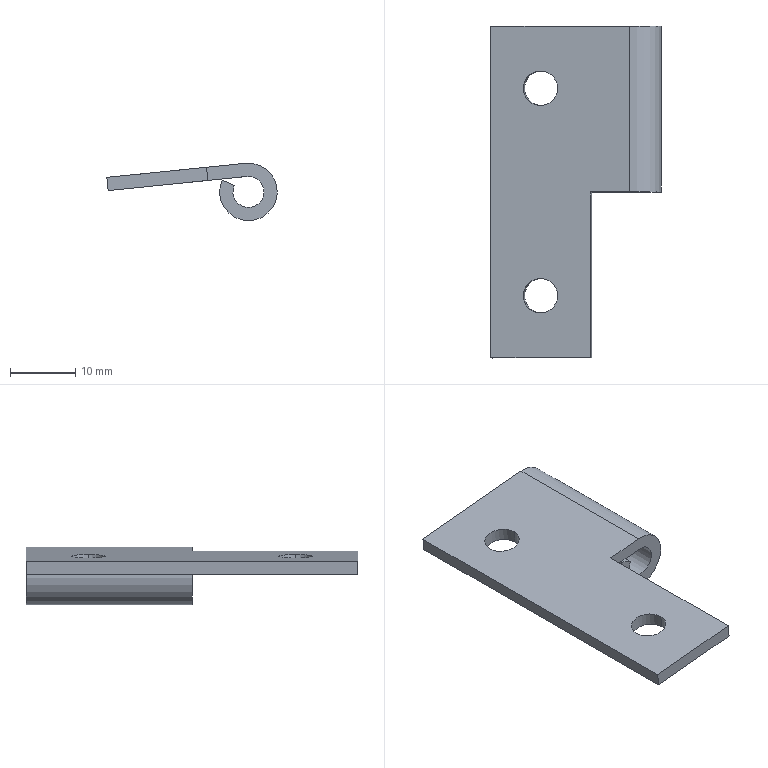Component | SolidWorks | Imported3-1 | 1 solid | 15 faces | box 26.08 x 50.8 x 8.81 mm | volume 2720 mm3 | plane 9 | cylinder 6 | commonest cylinder face diameters 5.283 x4 8.814 x1 4.75 x1
STEP:
#1=COLOUR_RGB('',0.7922,0.8196,0.9333);
#2=FILL_AREA_STYLE_COLOUR('',#1);
#3=FILL_AREA_STYLE('',(#2));
#4=SURFACE_STYLE_FILL_AREA(#3);
#5=SURFACE_SIDE_STYLE('',(#4));
#6=SURFACE_STYLE_USAGE(.BOTH.,#5);
#7=PRESENTATION_STYLE_ASSIGNMENT((#6));
#8=CARTESIAN_POINT('',(-8.855,6.998,9.99));
#9=VERTEX_POINT('',#8);
#10=CARTESIAN_POINT('',(-8.648,6.998,10.011));
#11=VERTEX_POINT('',#10);
#12=CARTESIAN_POINT('',(-8.751,6.998,10.001));
#13=DIRECTION('',(0.1012,0.,-0.9949));
#14=DIRECTION('',(-0.9949,0.,-0.1012));
#15=AXIS2_PLACEMENT_3D('',#12,#13,#14);
#16=CIRCLE('',#15,0.104);
#17=EDGE_CURVE('',#9,#11,#16,.T.);
#18=ORIENTED_EDGE('',*,*,#17,.F.);
#19=CARTESIAN_POINT('',(-8.847,6.998,9.91));
#20=VERTEX_POINT('',#19);
#21=CARTESIAN_POINT('',(-8.855,6.998,9.99));
#22=DIRECTION('',(0.1012,0.,-0.9949));
#23=VECTOR('',#22,39.37);
#24=LINE('',#21,#23);
#25=EDGE_CURVE('',#9,#20,#24,.T.);
#26=ORIENTED_EDGE('',*,*,#25,.T.);
#27=CARTESIAN_POINT('',(-8.64,6.998,9.931));
#28=VERTEX_POINT('',#27);
#29=CARTESIAN_POINT('',(-8.743,6.998,9.921));
#30=DIRECTION('',(0.1012,0.,-0.9949));
#31=DIRECTION('',(-0.9949,0.,-0.1012));
#32=AXIS2_PLACEMENT_3D('',#29,#30,#31);
#33=CIRCLE('',#32,0.104);
#34=EDGE_CURVE('',#20,#28,#33,.T.);
#35=ORIENTED_EDGE('',*,*,#34,.T.);
#36=CARTESIAN_POINT('',(-8.648,6.998,10.011));
#37=DIRECTION('',(0.1012,0.,-0.9949));
#38=VECTOR('',#37,39.37);
#39=LINE('',#36,#38);
#40=EDGE_CURVE('',#11,#28,#39,.T.);
#41=ORIENTED_EDGE('',*,*,#40,.F.);
#42=EDGE_LOOP('',(#18,#26,#35,#41));
#43=FACE_OUTER_BOUND('',#42,.T.);
#44=CARTESIAN_POINT('',(-8.751,6.998,10.001));
#45=DIRECTION('',(0.1012,0.,-0.9949));
#46=DIRECTION('',(0.9949,0.,0.1012));
#47=AXIS2_PLACEMENT_3D('',#44,#45,#46);
#48=CYLINDRICAL_SURFACE('',#47,0.104);
#49=ADVANCED_FACE('',(#43),#48,.F.);
#50=CARTESIAN_POINT('',(-8.855,5.748,9.99));
#51=VERTEX_POINT('',#50);
#52=CARTESIAN_POINT('',(-8.648,5.748,10.011));
#53=VERTEX_POINT('',#52);
#54=CARTESIAN_POINT('',(-8.751,5.748,10.001));
#55=DIRECTION('',(0.1012,0.,-0.9949));
#56=DIRECTION('',(0.9949,0.,0.1012));
#57=AXIS2_PLACEMENT_3D('',#54,#55,#56);
#58=CIRCLE('',#57,0.104);
#59=EDGE_CURVE('',#51,#53,#58,.T.);
#60=ORIENTED_EDGE('',*,*,#59,.F.);
#61=CARTESIAN_POINT('',(-8.847,5.748,9.91));
#62=VERTEX_POINT('',#61);
#63=CARTESIAN_POINT('',(-8.855,5.748,9.99));
#64=DIRECTION('',(0.1012,0.,-0.9949));
#65=VECTOR('',#64,39.37);
#66=LINE('',#63,#65);
#67=EDGE_CURVE('',#51,#62,#66,.T.);
#68=ORIENTED_EDGE('',*,*,#67,.T.);
#69=CARTESIAN_POINT('',(-8.64,5.748,9.931));
#70=VERTEX_POINT('',#69);
#71=CARTESIAN_POINT('',(-8.743,5.748,9.921));
#72=DIRECTION('',(0.1012,0.,-0.9949));
#73=DIRECTION('',(0.9949,0.,0.1012));
#74=AXIS2_PLACEMENT_3D('',#71,#72,#73);
#75=CIRCLE('',#74,0.104);
#76=EDGE_CURVE('',#62,#70,#75,.T.);
#77=ORIENTED_EDGE('',*,*,#76,.T.);
#78=CARTESIAN_POINT('',(-8.648,5.748,10.011));
#79=DIRECTION('',(0.1012,0.,-0.9949));
#80=VECTOR('',#79,39.37);
#81=LINE('',#78,#80);
#82=EDGE_CURVE('',#53,#70,#81,.T.);
#83=ORIENTED_EDGE('',*,*,#82,.F.);
#84=EDGE_LOOP('',(#60,#68,#77,#83));
#85=FACE_OUTER_BOUND('',#84,.T.);
#86=CARTESIAN_POINT('',(-8.751,5.748,10.001));
#87=DIRECTION('',(0.1012,0.,-0.9949));
#88=DIRECTION('',(0.9949,0.,0.1012));
#89=AXIS2_PLACEMENT_3D('',#86,#87,#88);
#90=CYLINDRICAL_SURFACE('',#89,0.104);
#91=ADVANCED_FACE('',(#85),#90,.F.);
#92=CARTESIAN_POINT('',(-9.05,5.373,9.97));
#93=VERTEX_POINT('',#92);
#94=CARTESIAN_POINT('',(-9.05,7.373,9.97));
#95=VERTEX_POINT('',#94);
#96=CARTESIAN_POINT('',(-9.05,5.373,9.97));
#97=DIRECTION('',(-0.,1.,0.));
#98=VECTOR('',#97,39.37);
#99=LINE('',#96,#98);
#100=EDGE_CURVE('',#93,#95,#99,.T.);
#101=ORIENTED_EDGE('',*,*,#100,.T.);
#102=CARTESIAN_POINT('',(-9.042,7.373,9.891));
#103=VERTEX_POINT('',#102);
#104=CARTESIAN_POINT('',(-9.042,7.373,9.891));
#105=DIRECTION('',(-0.1012,-0.,0.9949));
#106=VECTOR('',#105,39.37);
#107=LINE('',#104,#106);
#108=EDGE_CURVE('',#103,#95,#107,.T.);
#109=ORIENTED_EDGE('',*,*,#108,.F.);
#110=CARTESIAN_POINT('',(-9.042,5.373,9.891));
#111=VERTEX_POINT('',#110);
#112=CARTESIAN_POINT('',(-9.042,5.373,9.891));
#113=DIRECTION('',(-0.,1.,0.));
#114=VECTOR('',#113,39.37);
#115=LINE('',#112,#114);
#116=EDGE_CURVE('',#111,#103,#115,.T.);
#117=ORIENTED_EDGE('',*,*,#116,.F.);
#118=CARTESIAN_POINT('',(-9.042,5.373,9.891));
#119=DIRECTION('',(-0.1012,-0.,0.9949));
#120=VECTOR('',#119,39.37);
#121=LINE('',#118,#120);
#122=EDGE_CURVE('',#111,#93,#121,.T.);
#123=ORIENTED_EDGE('',*,*,#122,.T.);
#124=EDGE_LOOP('',(#101,#109,#117,#123));
#125=FACE_OUTER_BOUND('',#124,.T.);
#126=CARTESIAN_POINT('',(-9.042,5.373,9.891));
#127=DIRECTION('',(0.9949,0.,0.1012));
#128=DIRECTION('',(-0.1012,-0.,0.9949));
#129=AXIS2_PLACEMENT_3D('',#126,#127,#128);
#130=PLANE('',#129);
#131=ADVANCED_FACE('',(#125),#130,.F.);
#132=CARTESIAN_POINT('',(-8.214,7.373,10.055));
#133=VERTEX_POINT('',#132);
#134=CARTESIAN_POINT('',(-9.05,7.373,9.97));
#135=DIRECTION('',(0.9949,0.,0.1012));
#136=VECTOR('',#135,39.37);
#137=LINE('',#134,#136);
#138=EDGE_CURVE('',#95,#133,#137,.T.);
#139=ORIENTED_EDGE('',*,*,#138,.T.);
#140=CARTESIAN_POINT('',(-8.206,7.373,9.976));
#141=VERTEX_POINT('',#140);
#142=CARTESIAN_POINT('',(-8.206,7.373,9.976));
#143=DIRECTION('',(-0.1012,-0.,0.9949));
#144=VECTOR('',#143,39.37);
#145=LINE('',#142,#144);
#146=EDGE_CURVE('',#141,#133,#145,.T.);
#147=ORIENTED_EDGE('',*,*,#146,.F.);
#148=CARTESIAN_POINT('',(-9.042,7.373,9.891));
#149=DIRECTION('',(0.9949,0.,0.1012));
#150=VECTOR('',#149,39.37);
#151=LINE('',#148,#150);
#152=EDGE_CURVE('',#103,#141,#151,.T.);
#153=ORIENTED_EDGE('',*,*,#152,.F.);
#154=ORIENTED_EDGE('',*,*,#108,.T.);
#155=EDGE_LOOP('',(#139,#147,#153,#154));
#156=FACE_OUTER_BOUND('',#155,.T.);
#157=CARTESIAN_POINT('',(-9.042,7.373,9.891));
#158=DIRECTION('',(0.,-1.,-0.));
#159=DIRECTION('',(0.1012,0.,-0.9949));
#160=AXIS2_PLACEMENT_3D('',#157,#158,#159);
#161=PLANE('',#160);
#162=ADVANCED_FACE('',(#156),#161,.F.);
#163=CARTESIAN_POINT('',(-8.441,5.373,9.952));
#164=VERTEX_POINT('',#163);
#165=CARTESIAN_POINT('',(-9.042,5.373,9.891));
#166=DIRECTION('',(-0.9949,-0.,-0.1012));
#167=VECTOR('',#166,39.37);
#168=LINE('',#165,#167);
#169=EDGE_CURVE('',#164,#111,#168,.T.);
#170=ORIENTED_EDGE('',*,*,#169,.F.);
#171=CARTESIAN_POINT('',(-8.449,5.373,10.031));
#172=VERTEX_POINT('',#171);
#173=CARTESIAN_POINT('',(-8.414,5.373,9.686));
#174=DIRECTION('',(-0.1012,-0.,0.9949));
#175=VECTOR('',#174,39.37);
#176=LINE('',#173,#175);
#177=EDGE_CURVE('',#164,#172,#176,.T.);
#178=ORIENTED_EDGE('',*,*,#177,.T.);
#179=CARTESIAN_POINT('',(-9.05,5.373,9.97));
#180=DIRECTION('',(-0.9949,-0.,-0.1012));
#181=VECTOR('',#180,39.37);
#182=LINE('',#179,#181);
#183=EDGE_CURVE('',#172,#93,#182,.T.);
#184=ORIENTED_EDGE('',*,*,#183,.T.);
#185=ORIENTED_EDGE('',*,*,#122,.F.);
#186=EDGE_LOOP('',(#170,#178,#184,#185));
#187=FACE_OUTER_BOUND('',#186,.T.);
#188=CARTESIAN_POINT('',(-9.042,5.373,9.891));
#189=DIRECTION('',(-0.,1.,0.));
#190=DIRECTION('',(-0.1012,-0.,0.9949));
#191=AXIS2_PLACEMENT_3D('',#188,#189,#190);
#192=PLANE('',#191);
#193=ADVANCED_FACE('',(#187),#192,.F.);
#194=CARTESIAN_POINT('',(-8.743,6.998,9.921));
#195=DIRECTION('',(0.1012,0.,-0.9949));
#196=DIRECTION('',(-0.9949,0.,-0.1012));
#197=AXIS2_PLACEMENT_3D('',#194,#195,#196);
#198=CIRCLE('',#197,0.104);
#199=EDGE_CURVE('',#28,#20,#198,.T.);
#200=ORIENTED_EDGE('',*,*,#199,.F.);
#201=ORIENTED_EDGE('',*,*,#34,.F.);
#202=EDGE_LOOP('',(#200,#201));
#203=FACE_BOUND('',#202,.T.);
#204=CARTESIAN_POINT('',(-8.743,5.748,9.921));
#205=DIRECTION('',(0.1012,0.,-0.9949));
#206=DIRECTION('',(0.9949,0.,0.1012));
#207=AXIS2_PLACEMENT_3D('',#204,#205,#206);
#208=CIRCLE('',#207,0.104);
#209=EDGE_CURVE('',#70,#62,#208,.T.);
#210=ORIENTED_EDGE('',*,*,#209,.F.);
#211=ORIENTED_EDGE('',*,*,#76,.F.);
#212=EDGE_LOOP('',(#210,#211));
#213=FACE_BOUND('',#212,.T.);
#214=CARTESIAN_POINT('',(-8.441,6.373,9.952));
#215=VERTEX_POINT('',#214);
#216=CARTESIAN_POINT('',(-8.441,7.373,9.952));
#217=DIRECTION('',(-0.,1.,0.));
#218=VECTOR('',#217,39.37);
#219=LINE('',#216,#218);
#220=EDGE_CURVE('',#164,#215,#219,.T.);
#221=ORIENTED_EDGE('',*,*,#220,.F.);
#222=ORIENTED_EDGE('',*,*,#169,.T.);
#223=ORIENTED_EDGE('',*,*,#116,.T.);
#224=ORIENTED_EDGE('',*,*,#152,.T.);
#225=CARTESIAN_POINT('',(-8.206,6.373,9.976));
#226=VERTEX_POINT('',#225);
#227=CARTESIAN_POINT('',(-8.206,5.373,9.976));
#228=DIRECTION('',(0.,-1.,-0.));
#229=VECTOR('',#228,39.37);
#230=LINE('',#227,#229);
#231=EDGE_CURVE('',#141,#226,#230,.T.);
#232=ORIENTED_EDGE('',*,*,#231,.T.);
#233=CARTESIAN_POINT('',(-9.042,6.373,9.891));
#234=DIRECTION('',(0.9949,0.,0.1012));
#235=VECTOR('',#234,39.37);
#236=LINE('',#233,#235);
#237=EDGE_CURVE('',#215,#226,#236,.T.);
#238=ORIENTED_EDGE('',*,*,#237,.F.);
#239=EDGE_LOOP('',(#221,#222,#223,#224,#232,#238));
#240=FACE_OUTER_BOUND('',#239,.T.);
#241=CARTESIAN_POINT('',(-9.042,7.373,9.891));
#242=DIRECTION('',(0.1012,0.,-0.9949));
#243=DIRECTION('',(0.9949,0.,0.1012));
#244=AXIS2_PLACEMENT_3D('',#241,#242,#243);
#245=PLANE('',#244);
#246=ADVANCED_FACE('',(#203,#213,#240),#245,.T.);
#247=CARTESIAN_POINT('',(-8.751,6.998,10.001));
#248=DIRECTION('',(0.1012,0.,-0.9949));
#249=DIRECTION('',(-0.9949,0.,-0.1012));
#250=AXIS2_PLACEMENT_3D('',#247,#248,#249);
#251=CIRCLE('',#250,0.104);
#252=EDGE_CURVE('',#11,#9,#251,.T.);
#253=ORIENTED_EDGE('',*,*,#252,.T.);
#254=ORIENTED_EDGE('',*,*,#17,.T.);
#255=EDGE_LOOP('',(#253,#254));
#256=FACE_BOUND('',#255,.T.);
#257=CARTESIAN_POINT('',(-8.751,5.748,10.001));
#258=DIRECTION('',(0.1012,0.,-0.9949));
#259=DIRECTION('',(0.9949,0.,0.1012));
#260=AXIS2_PLACEMENT_3D('',#257,#258,#259);
#261=CIRCLE('',#260,0.104);
#262=EDGE_CURVE('',#53,#51,#261,.T.);
#263=ORIENTED_EDGE('',*,*,#262,.T.);
#264=ORIENTED_EDGE('',*,*,#59,.T.);
#265=EDGE_LOOP('',(#263,#264));
#266=FACE_BOUND('',#265,.T.);
#267=ORIENTED_EDGE('',*,*,#183,.F.);
#268=CARTESIAN_POINT('',(-8.449,6.373,10.031));
#269=VERTEX_POINT('',#268);
#270=CARTESIAN_POINT('',(-8.449,5.373,10.031));
#271=DIRECTION('',(0.,-1.,-0.));
#272=VECTOR('',#271,39.37);
#273=LINE('',#270,#272);
#274=EDGE_CURVE('',#269,#172,#273,.T.);
#275=ORIENTED_EDGE('',*,*,#274,.F.);
#276=CARTESIAN_POINT('',(-8.214,6.373,10.055));
#277=VERTEX_POINT('',#276);
#278=CARTESIAN_POINT('',(-8.041,6.373,10.073));
#279=DIRECTION('',(-0.9949,-0.,-0.1012));
#280=VECTOR('',#279,39.37);
#281=LINE('',#278,#280);
#282=EDGE_CURVE('',#277,#269,#281,.T.);
#283=ORIENTED_EDGE('',*,*,#282,.F.);
#284=CARTESIAN_POINT('',(-8.214,5.373,10.055));
#285=DIRECTION('',(0.,-1.,-0.));
#286=VECTOR('',#285,39.37);
#287=LINE('',#284,#286);
#288=EDGE_CURVE('',#133,#277,#287,.T.);
#289=ORIENTED_EDGE('',*,*,#288,.F.);
#290=ORIENTED_EDGE('',*,*,#138,.F.);
#291=ORIENTED_EDGE('',*,*,#100,.F.);
#292=EDGE_LOOP('',(#267,#275,#283,#289,#290,#291));
#293=FACE_OUTER_BOUND('',#292,.T.);
#294=CARTESIAN_POINT('',(-9.05,7.373,9.97));
#295=DIRECTION('',(0.1012,0.,-0.9949));
#296=DIRECTION('',(0.9949,0.,0.1012));
#297=AXIS2_PLACEMENT_3D('',#294,#295,#296);
#298=PLANE('',#297);
#299=ADVANCED_FACE('',(#256,#266,#293),#298,.F.);
#300=CARTESIAN_POINT('',(-8.282,6.373,9.921));
#301=VERTEX_POINT('',#300);
#302=CARTESIAN_POINT('',(-8.355,6.373,9.954));
#303=VERTEX_POINT('',#302);
#304=CARTESIAN_POINT('',(-8.282,6.373,9.921));
#305=DIRECTION('',(-0.9122,-0.,0.4098));
#306=VECTOR('',#305,39.37);
#307=LINE('',#304,#306);
#308=EDGE_CURVE('',#301,#303,#307,.T.);
#309=ORIENTED_EDGE('',*,*,#308,.F.);
#310=CARTESIAN_POINT('',(-8.282,7.373,9.921));
#311=VERTEX_POINT('',#310);
#312=CARTESIAN_POINT('',(-8.282,5.373,9.921));
#313=DIRECTION('',(0.,-1.,-0.));
#314=VECTOR('',#313,39.37);
#315=LINE('',#312,#314);
#316=EDGE_CURVE('',#311,#301,#315,.T.);
#317=ORIENTED_EDGE('',*,*,#316,.F.);
#318=CARTESIAN_POINT('',(-8.355,7.373,9.954));
#319=VERTEX_POINT('',#318);
#320=CARTESIAN_POINT('',(-8.282,7.373,9.921));
#321=DIRECTION('',(-0.9122,-0.,0.4098));
#322=VECTOR('',#321,39.37);
#323=LINE('',#320,#322);
#324=EDGE_CURVE('',#311,#319,#323,.T.);
#325=ORIENTED_EDGE('',*,*,#324,.T.);
#326=CARTESIAN_POINT('',(-8.355,5.373,9.954));
#327=DIRECTION('',(0.,-1.,-0.));
#328=VECTOR('',#327,39.37);
#329=LINE('',#326,#328);
#330=EDGE_CURVE('',#319,#303,#329,.T.);
#331=ORIENTED_EDGE('',*,*,#330,.T.);
#332=EDGE_LOOP('',(#309,#317,#325,#331));
#333=FACE_OUTER_BOUND('',#332,.T.);
#334=CARTESIAN_POINT('',(-8.282,6.373,9.921));
#335=DIRECTION('',(-0.4098,0.,-0.9122));
#336=DIRECTION('',(0.,-1.,-0.));
#337=AXIS2_PLACEMENT_3D('',#334,#335,#336);
#338=PLANE('',#337);
#339=ADVANCED_FACE('',(#333),#338,.F.);
#340=ORIENTED_EDGE('',*,*,#324,.F.);
#341=CARTESIAN_POINT('',(-8.196,7.373,9.883));
#342=DIRECTION('',(-0.,1.,0.));
#343=DIRECTION('',(0.1012,0.,-0.9949));
#344=AXIS2_PLACEMENT_3D('',#341,#342,#343);
#345=CIRCLE('',#344,0.0935);
#346=EDGE_CURVE('',#141,#311,#345,.T.);
#347=ORIENTED_EDGE('',*,*,#346,.F.);
#348=ORIENTED_EDGE('',*,*,#146,.T.);
#349=CARTESIAN_POINT('',(-8.196,7.373,9.883));
#350=DIRECTION('',(-0.,1.,0.));
#351=DIRECTION('',(0.1012,0.,-0.9949));
#352=AXIS2_PLACEMENT_3D('',#349,#350,#351);
#353=CIRCLE('',#352,0.1735);
#354=EDGE_CURVE('',#133,#319,#353,.T.);
#355=ORIENTED_EDGE('',*,*,#354,.T.);
#356=EDGE_LOOP('',(#340,#347,#348,#355));
#357=FACE_OUTER_BOUND('',#356,.T.);
#358=CARTESIAN_POINT('',(-8.196,7.373,9.883));
#359=DIRECTION('',(-0.,1.,0.));
#360=DIRECTION('',(-0.1012,-0.,0.9949));
#361=AXIS2_PLACEMENT_3D('',#358,#359,#360);
#362=PLANE('',#361);
#363=ADVANCED_FACE('',(#357),#362,.T.);
#364=CARTESIAN_POINT('',(-8.196,6.373,9.883));
#365=DIRECTION('',(0.,-1.,-0.));
#366=DIRECTION('',(0.9949,0.,0.1012));
#367=AXIS2_PLACEMENT_3D('',#364,#365,#366);
#368=CIRCLE('',#367,0.1735);
#369=EDGE_CURVE('',#303,#277,#368,.T.);
#370=ORIENTED_EDGE('',*,*,#369,.F.);
#371=ORIENTED_EDGE('',*,*,#330,.F.);
#372=ORIENTED_EDGE('',*,*,#354,.F.);
#373=ORIENTED_EDGE('',*,*,#288,.T.);
#374=EDGE_LOOP('',(#370,#371,#372,#373));
#375=FACE_OUTER_BOUND('',#374,.T.);
#376=CARTESIAN_POINT('',(-8.196,5.373,9.883));
#377=DIRECTION('',(0.,-1.,-0.));
#378=DIRECTION('',(-0.9122,0.,0.4098));
#379=AXIS2_PLACEMENT_3D('',#376,#377,#378);
#380=CYLINDRICAL_SURFACE('',#379,0.1735);
#381=ADVANCED_FACE('',(#375),#380,.T.);
#382=ORIENTED_EDGE('',*,*,#316,.T.);
#383=CARTESIAN_POINT('',(-8.196,6.373,9.883));
#384=DIRECTION('',(0.,-1.,-0.));
#385=DIRECTION('',(0.9949,0.,0.1012));
#386=AXIS2_PLACEMENT_3D('',#383,#384,#385);
#387=CIRCLE('',#386,0.0935);
#388=EDGE_CURVE('',#301,#226,#387,.T.);
#389=ORIENTED_EDGE('',*,*,#388,.T.);
#390=ORIENTED_EDGE('',*,*,#231,.F.);
#391=ORIENTED_EDGE('',*,*,#346,.T.);
#392=EDGE_LOOP('',(#382,#389,#390,#391));
#393=FACE_OUTER_BOUND('',#392,.T.);
#394=CARTESIAN_POINT('',(-8.196,5.373,9.883));
#395=DIRECTION('',(0.,-1.,-0.));
#396=DIRECTION('',(-0.9122,0.,0.4098));
#397=AXIS2_PLACEMENT_3D('',#394,#395,#396);
#398=CYLINDRICAL_SURFACE('',#397,0.0935);
#399=ADVANCED_FACE('',(#393),#398,.F.);
#400=ORIENTED_EDGE('',*,*,#220,.T.);
#401=CARTESIAN_POINT('',(-8.414,6.373,9.686));
#402=DIRECTION('',(-0.1012,-0.,0.9949));
#403=VECTOR('',#402,39.37);
#404=LINE('',#401,#403);
#405=EDGE_CURVE('',#215,#269,#404,.T.);
#406=ORIENTED_EDGE('',*,*,#405,.T.);
#407=ORIENTED_EDGE('',*,*,#274,.T.);
#408=ORIENTED_EDGE('',*,*,#177,.F.);
#409=EDGE_LOOP('',(#400,#406,#407,#408));
#410=FACE_OUTER_BOUND('',#409,.T.);
#411=CARTESIAN_POINT('',(-8.414,5.373,9.686));
#412=DIRECTION('',(-0.9949,-0.,-0.1012));
#413=DIRECTION('',(-0.,1.,0.));
#414=AXIS2_PLACEMENT_3D('',#411,#412,#413);
#415=PLANE('',#414);
#416=ADVANCED_FACE('',(#410),#415,.F.);
#417=ORIENTED_EDGE('',*,*,#369,.T.);
#418=ORIENTED_EDGE('',*,*,#282,.T.);
#419=ORIENTED_EDGE('',*,*,#405,.F.);
#420=ORIENTED_EDGE('',*,*,#237,.T.);
#421=ORIENTED_EDGE('',*,*,#388,.F.);
#422=ORIENTED_EDGE('',*,*,#308,.T.);
#423=EDGE_LOOP('',(#417,#418,#419,#420,#421,#422));
#424=FACE_OUTER_BOUND('',#423,.T.);
#425=CARTESIAN_POINT('',(-8.006,6.373,9.728));
#426=DIRECTION('',(-0.,1.,0.));
#427=DIRECTION('',(0.9949,0.,0.1012));
#428=AXIS2_PLACEMENT_3D('',#425,#426,#427);
#429=PLANE('',#428);
#430=ADVANCED_FACE('',(#424),#429,.F.);
#431=ORIENTED_EDGE('',*,*,#67,.F.);
#432=ORIENTED_EDGE('',*,*,#262,.F.);
#433=ORIENTED_EDGE('',*,*,#82,.T.);
#434=ORIENTED_EDGE('',*,*,#209,.T.);
#435=EDGE_LOOP('',(#431,#432,#433,#434));
#436=FACE_OUTER_BOUND('',#435,.T.);
#437=CARTESIAN_POINT('',(-8.751,5.748,10.001));
#438=DIRECTION('',(0.1012,0.,-0.9949));
#439=DIRECTION('',(0.9949,0.,0.1012));
#440=AXIS2_PLACEMENT_3D('',#437,#438,#439);
#441=CYLINDRICAL_SURFACE('',#440,0.104);
#442=ADVANCED_FACE('',(#436),#441,.F.);
#443=ORIENTED_EDGE('',*,*,#25,.F.);
#444=ORIENTED_EDGE('',*,*,#252,.F.);
#445=ORIENTED_EDGE('',*,*,#40,.T.);
#446=ORIENTED_EDGE('',*,*,#199,.T.);
#447=EDGE_LOOP('',(#443,#444,#445,#446));
#448=FACE_OUTER_BOUND('',#447,.T.);
#449=CARTESIAN_POINT('',(-8.751,6.998,10.001));
#450=DIRECTION('',(0.1012,0.,-0.9949));
#451=DIRECTION('',(0.9949,0.,0.1012));
#452=AXIS2_PLACEMENT_3D('',#449,#450,#451);
#453=CYLINDRICAL_SURFACE('',#452,0.104);
#454=ADVANCED_FACE('',(#448),#453,.F.);
#455=CLOSED_SHELL('',(#49,#91,#131,#162,#193,#246,#299,#339,#363,#381,#399,#416,#430,#442,#454));
#456=MANIFOLD_SOLID_BREP('',#455);
#457=STYLED_ITEM('',(#7),#456);
#458=(LENGTH_UNIT()NAMED_UNIT(*)SI_UNIT($,.METRE.));
#459=LENGTH_MEASURE_WITH_UNIT(LENGTH_MEASURE(0.0254),#458);
#460=DIMENSIONAL_EXPONENTS(1.,0.,0.,0.,0.,0.,0.);
#461=(CONVERSION_BASED_UNIT('',#459)LENGTH_UNIT()NAMED_UNIT(#460));
#462=UNCERTAINTY_MEASURE_WITH_UNIT(LENGTH_MEASURE(0.00001),#461,'','');
#463=(NAMED_UNIT(*)PLANE_ANGLE_UNIT()SI_UNIT($,.RADIAN.));
#464=(NAMED_UNIT(*)SI_UNIT($,.STERADIAN.)SOLID_ANGLE_UNIT());
#465=(GEOMETRIC_REPRESENTATION_CONTEXT(3)GLOBAL_UNCERTAINTY_ASSIGNED_CONTEXT((#462))GLOBAL_UNIT_ASSIGNED_CONTEXT((#461,#463,#464))REPRESENTATION_CONTEXT('',''));
#466=MECHANICAL_DESIGN_GEOMETRIC_PRESENTATION_REPRESENTATION('',(#457),#465);
#467=CARTESIAN_POINT('',(0.,0.,0.));
#468=DIRECTION('',(0.,0.,1.));
#469=DIRECTION('',(1.,0.,0.));
#470=AXIS2_PLACEMENT_3D('',#467,#468,#469);
#471=(LENGTH_UNIT()NAMED_UNIT(*)SI_UNIT($,.METRE.));
#472=LENGTH_MEASURE_WITH_UNIT(LENGTH_MEASURE(0.0254),#471);
#473=DIMENSIONAL_EXPONENTS(1.,0.,0.,0.,0.,0.,0.);
#474=(CONVERSION_BASED_UNIT('',#472)LENGTH_UNIT()NAMED_UNIT(#473));
#475=UNCERTAINTY_MEASURE_WITH_UNIT(LENGTH_MEASURE(0.00001),#474,'','');
#476=(NAMED_UNIT(*)PLANE_ANGLE_UNIT()SI_UNIT($,.RADIAN.));
#477=(NAMED_UNIT(*)SI_UNIT($,.STERADIAN.)SOLID_ANGLE_UNIT());
#478=(GEOMETRIC_REPRESENTATION_CONTEXT(3)GLOBAL_UNCERTAINTY_ASSIGNED_CONTEXT((#475))GLOBAL_UNIT_ASSIGNED_CONTEXT((#474,#476,#477))REPRESENTATION_CONTEXT('',''));
#479=ADVANCED_BREP_SHAPE_REPRESENTATION('',(#456,#470),#478);
#480=PRESENTATION_LAYER_ASSIGNMENT('','',(#457));